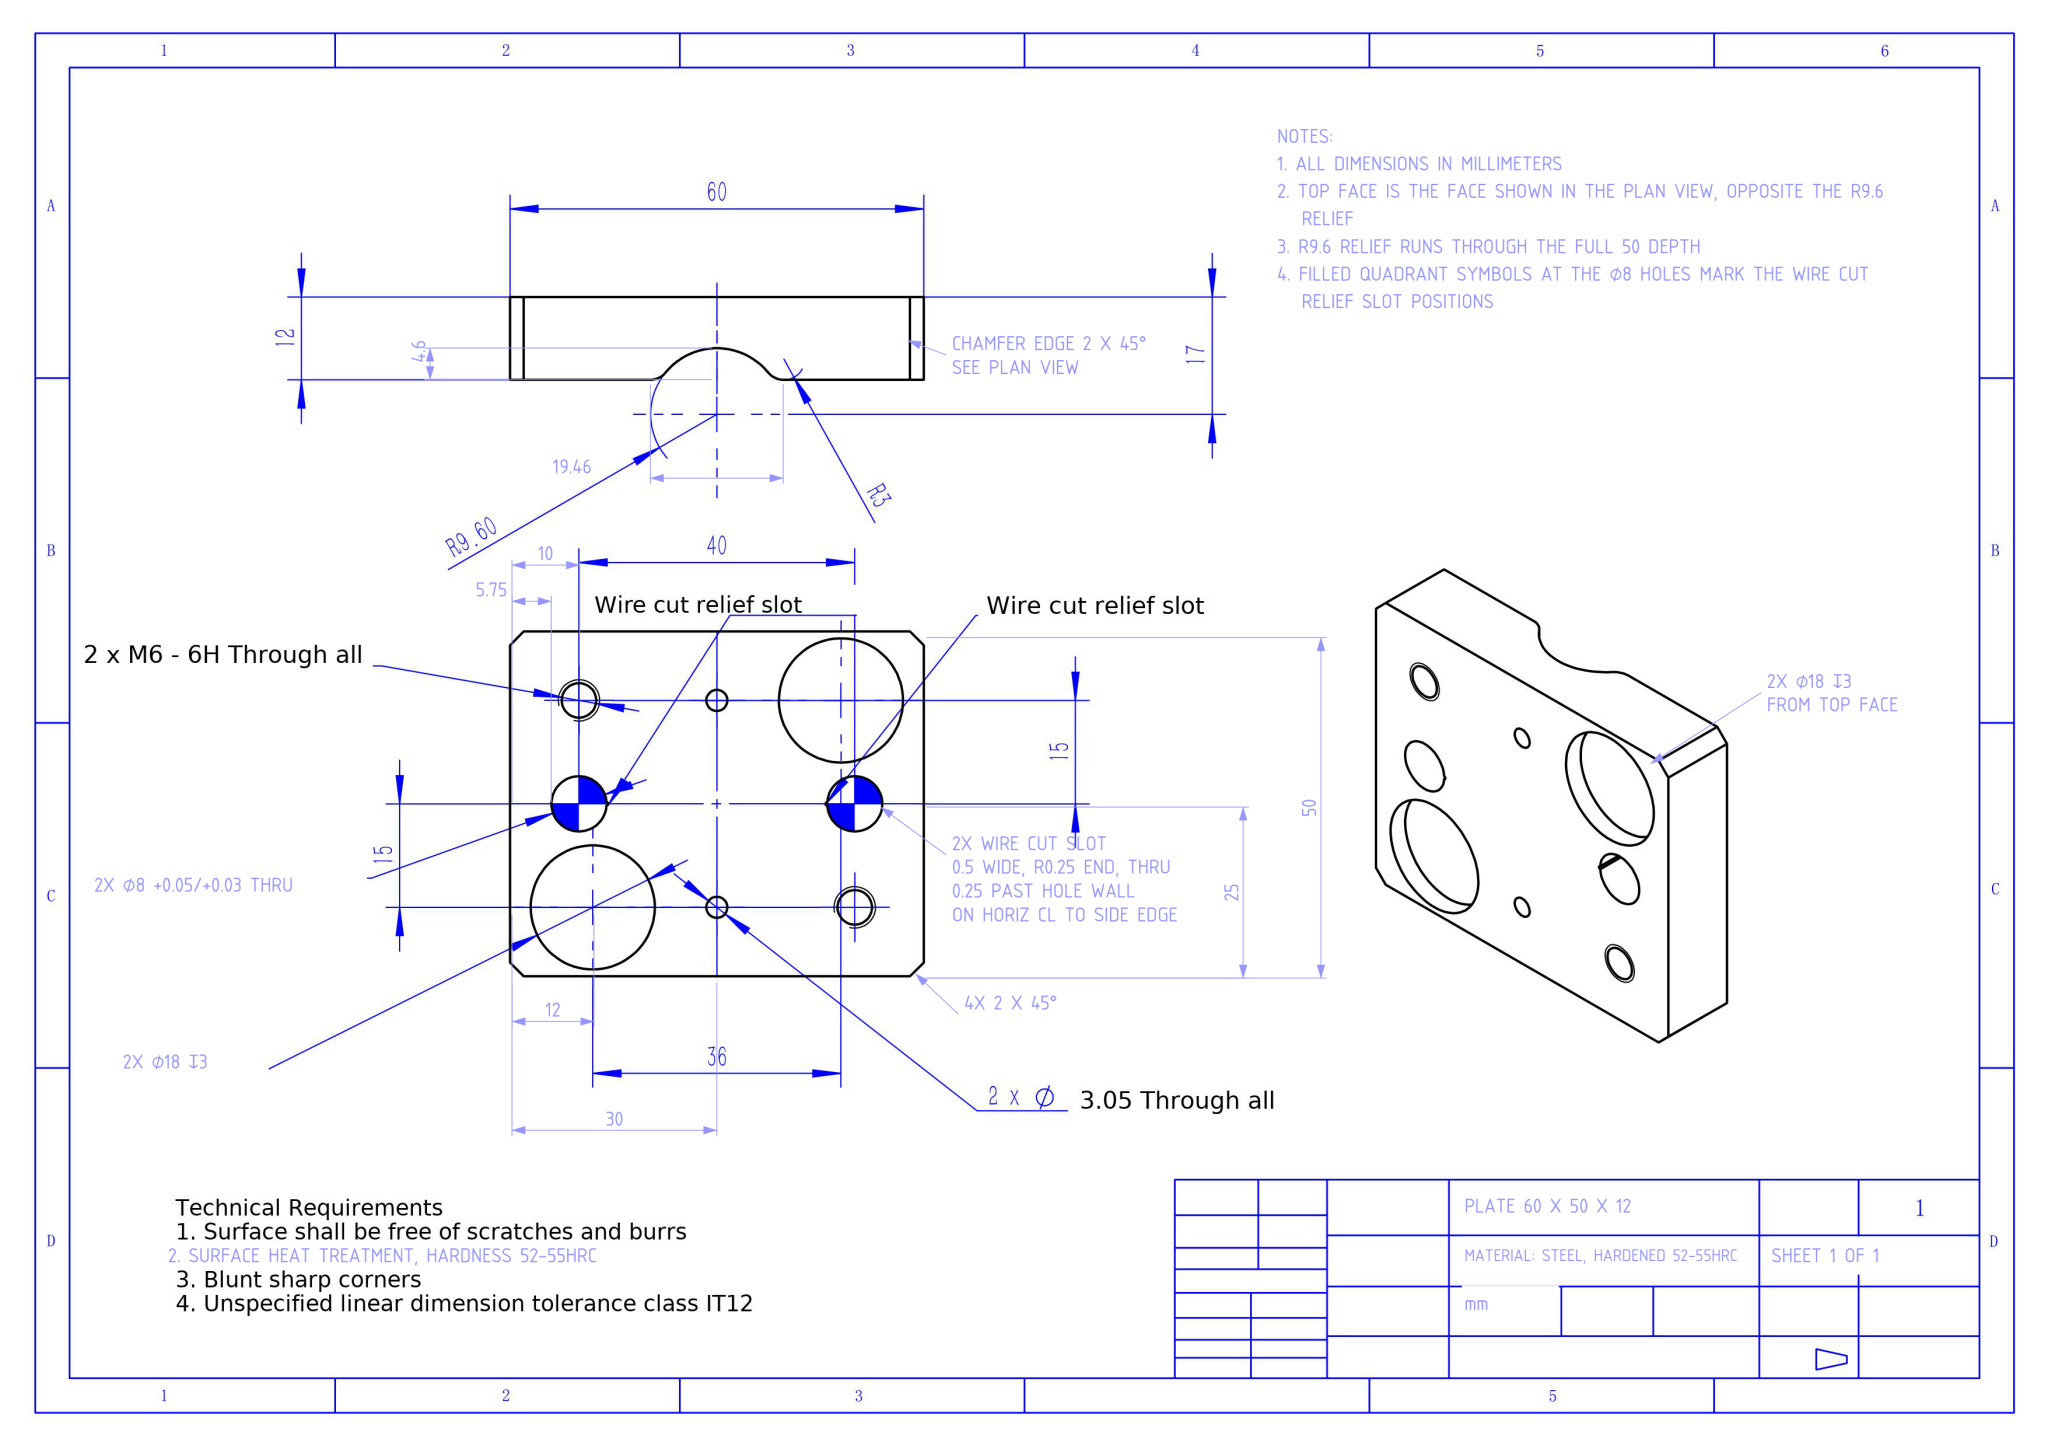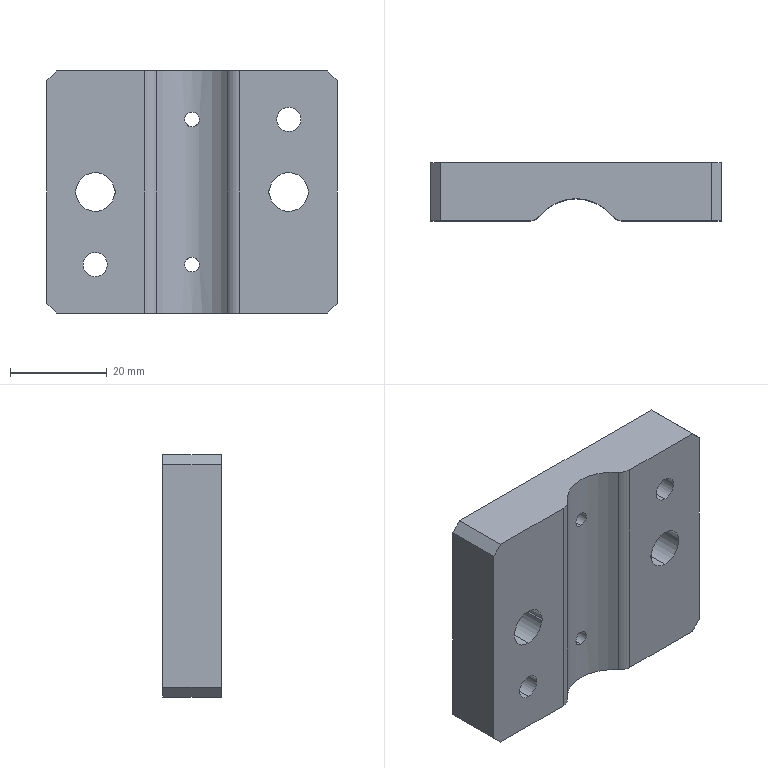Part | NX | mm | 1 solid | 40 faces | box 60 x 12 x 50 mm | volume 29891 mm3 | cylinder 27 | plane 13 | commonest cylinder face diameters 0.5 x6 8 x6 18 x4 5 x4 3.05 x4 6 x2 19.2 x1